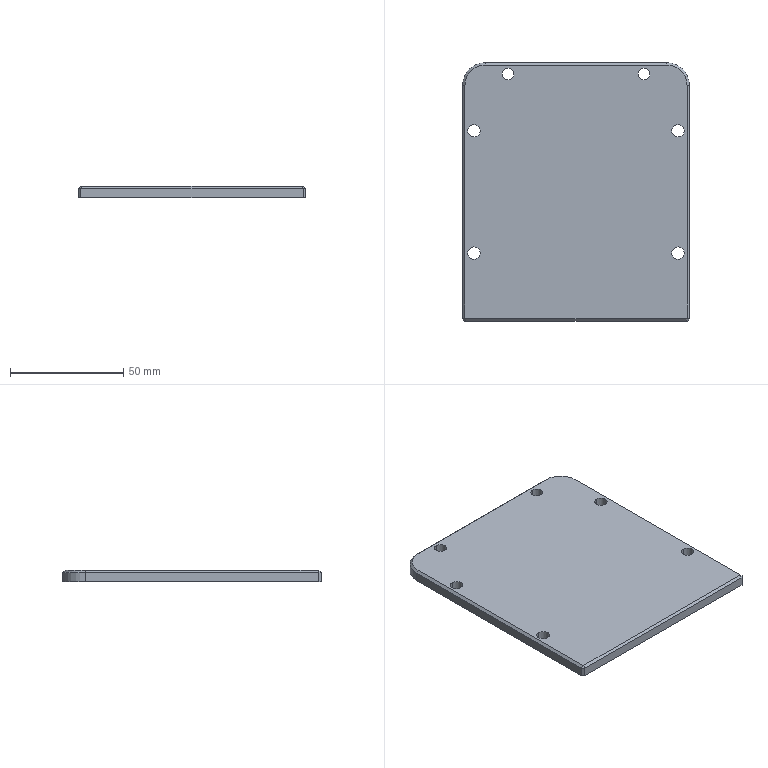CAM job | Mastercam | mm | 8 operations | part box 100 x 114 x 5
1. Facing | 24 - 100 平铣刀
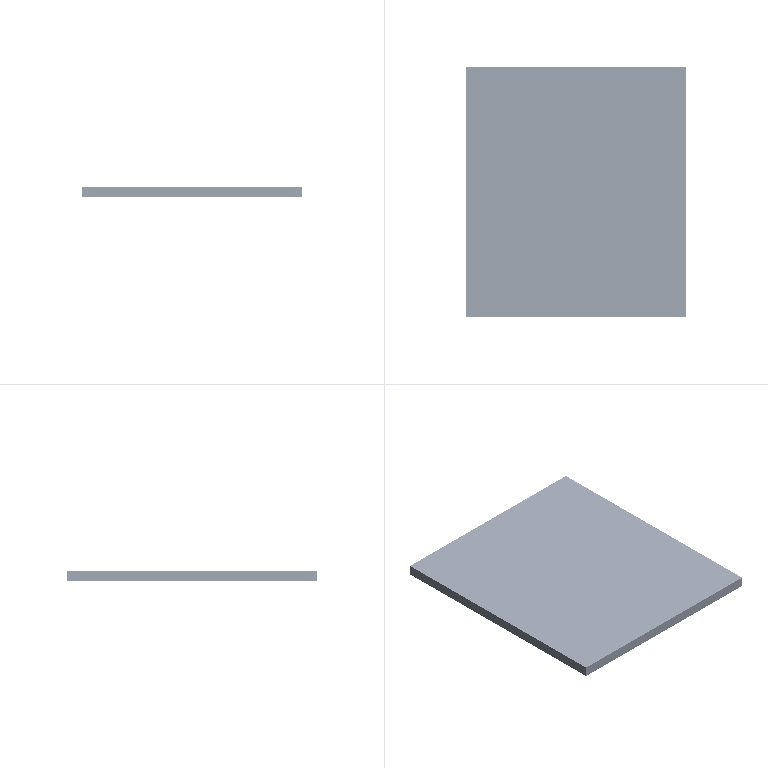2. 2D High Speed (2D Dynamic Mill) | 10 - 10 平铣刀
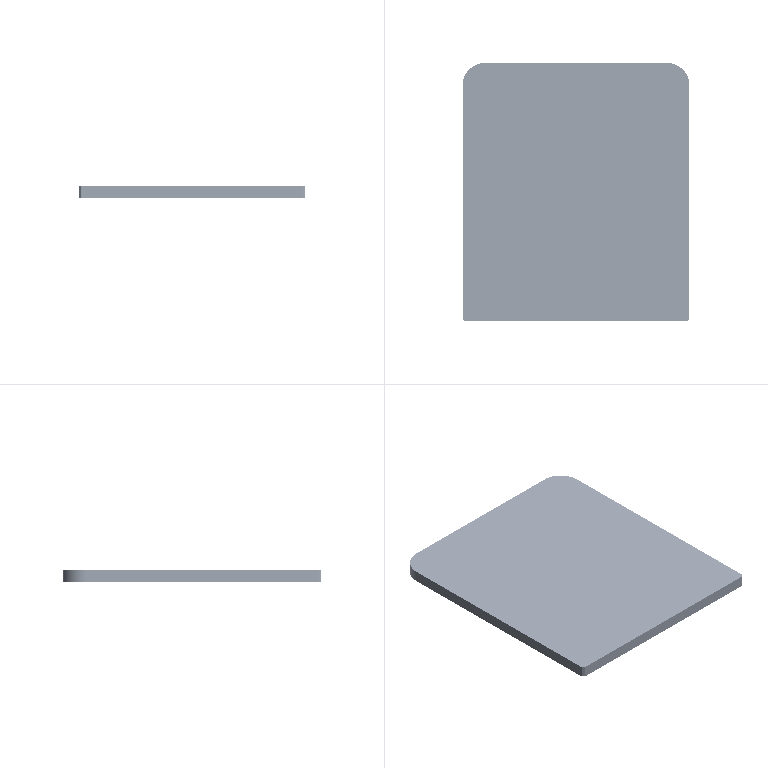3. Contour (2D) | 10 - 10 平铣刀
4. Drill/Counterbore | 7 - 4 倒角刀
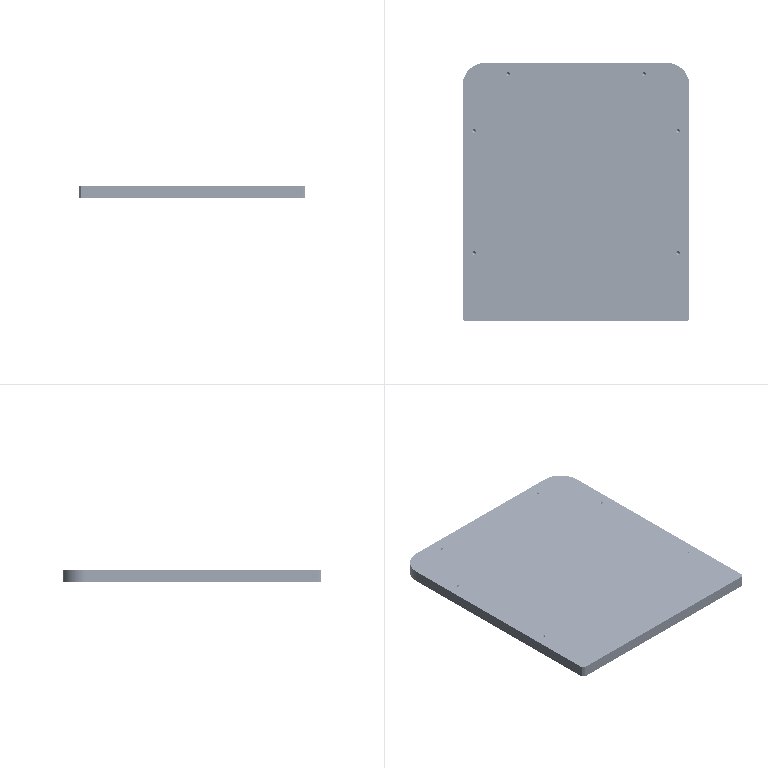5. Contour (2D chamfer) | 7 - 4 倒角刀
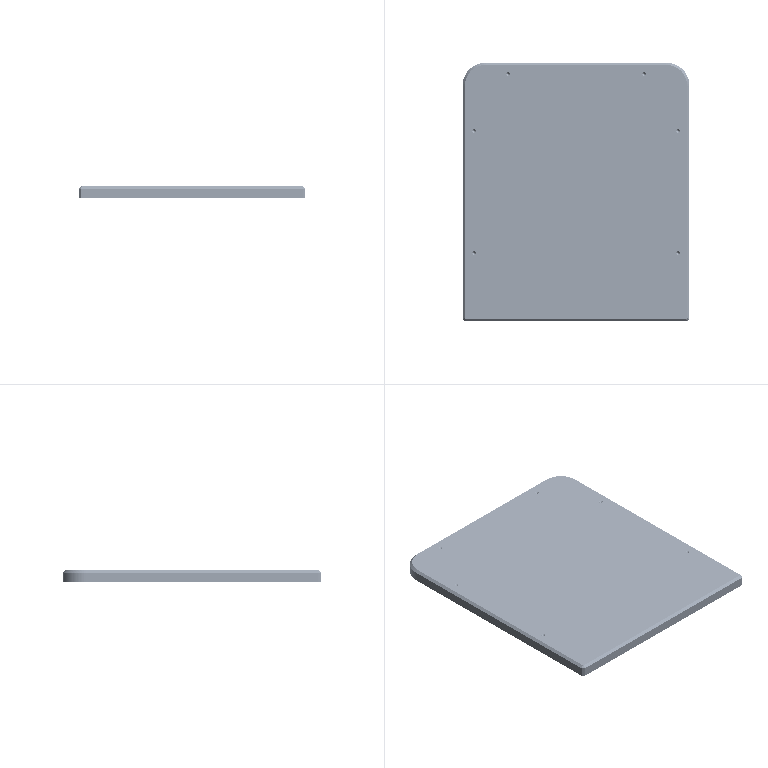6. Facing | 10 - 10 平铣刀
7. Facing | 24 - 100 平铣刀
8. Contour (2D chamfer) | 7 - 4 倒角刀